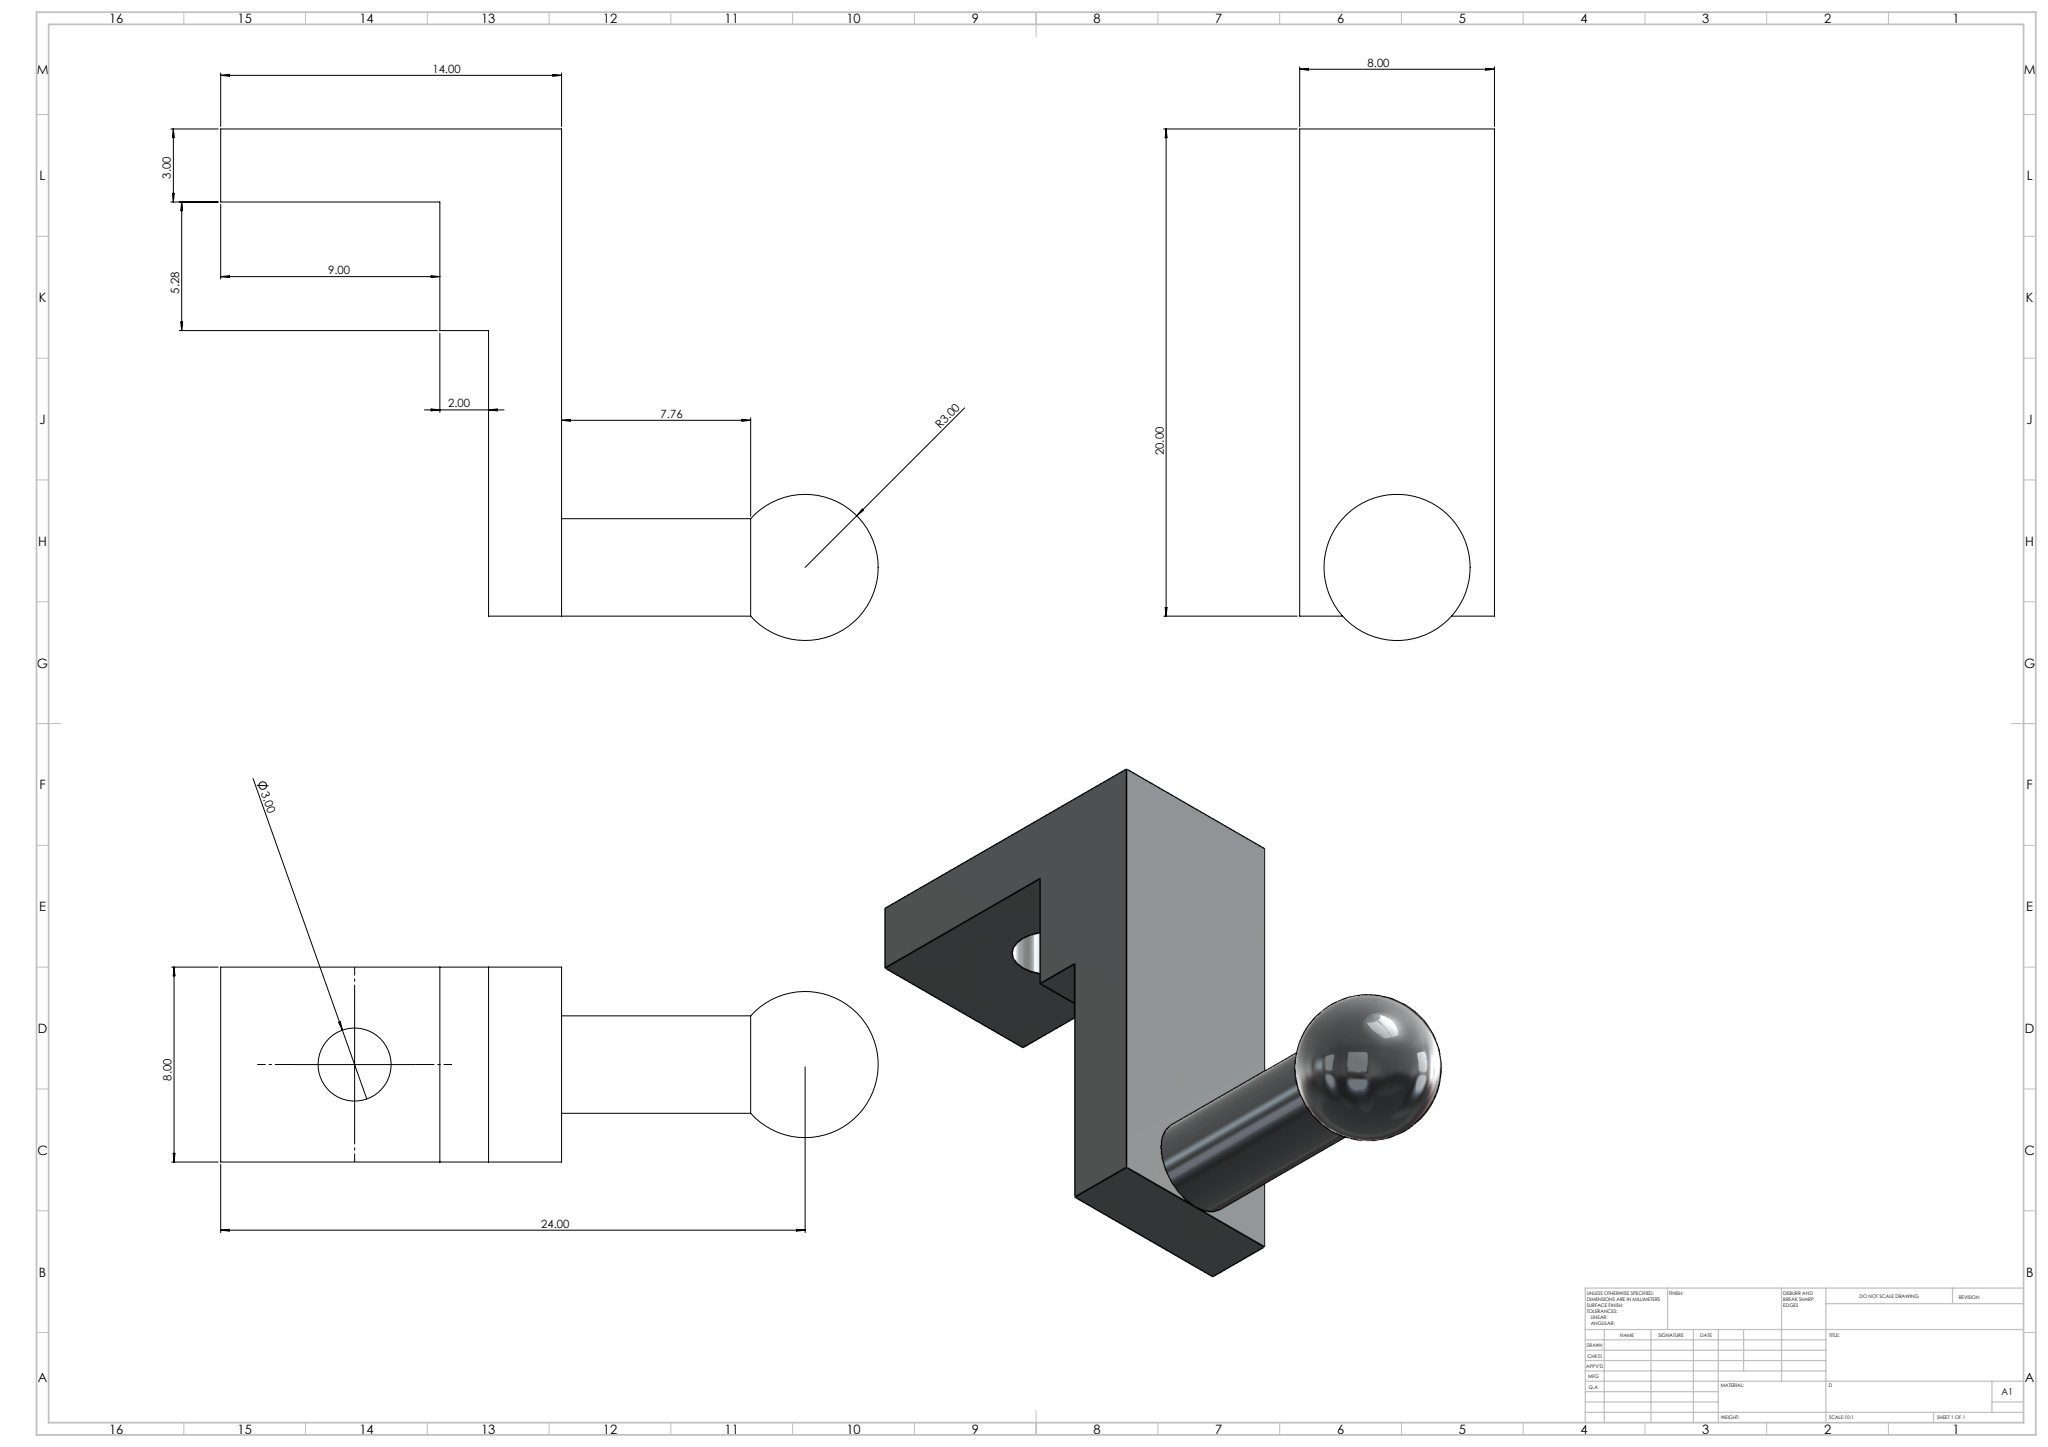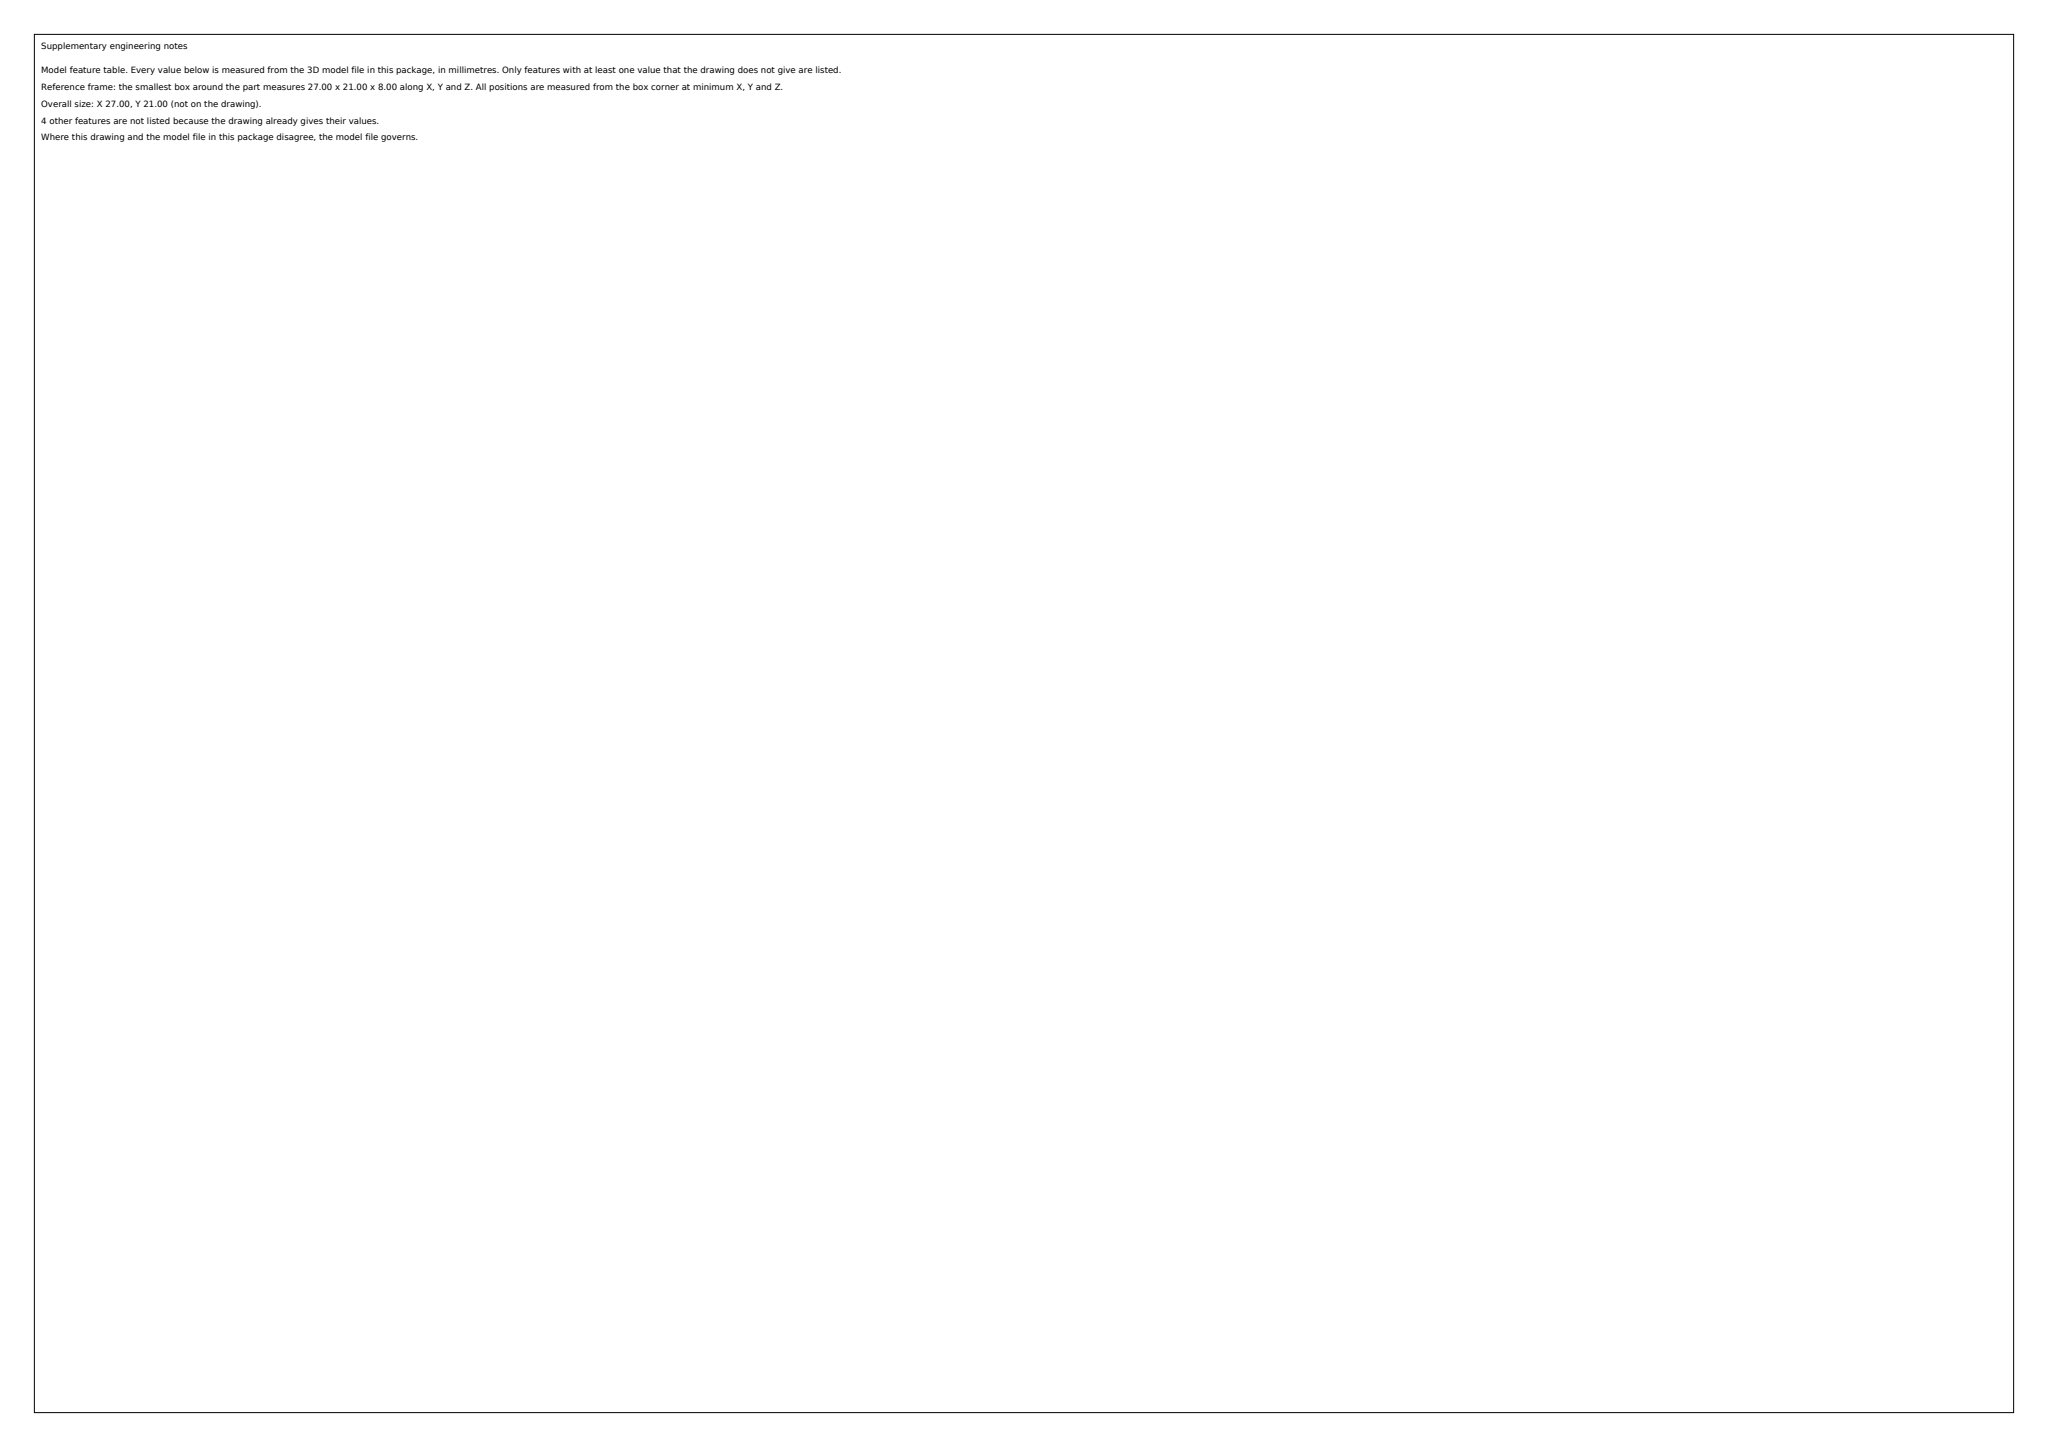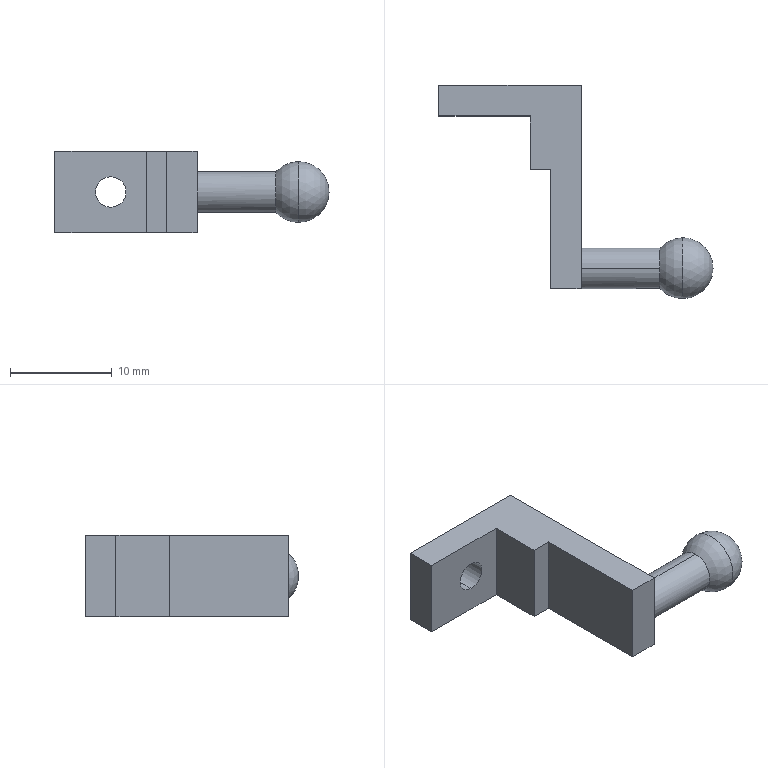Part | SolidWorks | mm | 1 solid | 16 faces | box 27 x 21 x 8 mm | volume 1013 mm3 | plane 10 | cylinder 4 | sphere 2 | commonest cylinder face diameters 3 x2 4 x2
build123d program:
from build123d import *

# Parameters (mm, degrees)
BOSS_EXTRUDE1_DEPTH = 8
SKETCH2_R           = 2
BOSS_EXTRUDE2_DEPTH = 10
CUT_EXTRUDE1_REACH  = 32.266
SKETCH4_R           = 1.5


with BuildPart() as part:
    # Sketch1 → Boss-Extrude1 (new body)
    with BuildSketch(Plane.XY):
        Polygon((-6.727, 7.437), (2.273, 7.437), (2.273, 2.159), (4.273, 2.159), (4.273, -9.563), (7.273, -9.563), (7.273, 10.437), (-6.727, 10.437), align=None)
    extrude(amount=BOSS_EXTRUDE1_DEPTH)

    # Sketch2 → Boss-Extrude2 (add)
    with BuildSketch(Plane(origin=(7.273, 0, 0), x_dir=(0, 0, -1), z_dir=(1, 0, 0))):
        with Locations(Location((-4, -7.563, 0), (0, 0, 270))):
            Circle(SKETCH2_R)
    extrude(amount=BOSS_EXTRUDE2_DEPTH)

    # Sketch3 → Revolve1 (revolve)
    with BuildSketch(Plane(origin=(17.273, 0, 0), x_dir=(0, 0, -1), z_dir=(1, 0, 0))):
        with BuildLine():
            Line((-7, -7.563), (-1, -7.563))
            ThreePointArc((-1, -7.563), (-4, -4.563), (-7, -7.563))
        make_face()
    revolve(axis=Axis((17.273, -7.563, 7), (0, 0, -1)))

    # Sketch4 → Cut-Extrude1 (cut, up to next)
    with BuildSketch(Plane(origin=(0, 10.437, 0), x_dir=(1, 0, 0), z_dir=(0, 1, 0)), mode=Mode.PRIVATE) as cut_extrude1_sk1:
        with Locations(Location((-1.227, -4, 0), (0, 0, 270))):
            Circle(SKETCH4_R)
    cut_extrude1_tool1 = extrude(cut_extrude1_sk1.sketch, amount=-CUT_EXTRUDE1_REACH, mode=Mode.PRIVATE) & part.part
    add(cut_extrude1_tool1.solids().sort_by_distance((-1.227, 10.437, 4))[0], mode=Mode.SUBTRACT)


solid = part.part
STEP:
#1=CARTESIAN_POINT('',(-1.227,7.437,5.5));
#2=VERTEX_POINT('',#1);
#3=CARTESIAN_POINT('',(-1.227,7.437,2.5));
#4=VERTEX_POINT('',#3);
#5=CARTESIAN_POINT('',(-1.227,7.437,4.));
#6=DIRECTION('',(0.,-1.,0.));
#7=DIRECTION('',(0.,0.,1.));
#8=AXIS2_PLACEMENT_3D('',#5,#6,#7);
#9=CIRCLE('',#8,1.5);
#10=EDGE_CURVE('',#2,#4,#9,.T.);
#11=ORIENTED_EDGE('',*,*,#10,.T.);
#12=CARTESIAN_POINT('',(-1.227,10.437,2.5));
#13=VERTEX_POINT('',#12);
#14=CARTESIAN_POINT('',(-1.227,-10.564,2.5));
#15=DIRECTION('',(0.,1.,0.));
#16=VECTOR('',#15,1000.);
#17=LINE('',#14,#16);
#18=EDGE_CURVE('',#4,#13,#17,.T.);
#19=ORIENTED_EDGE('',*,*,#18,.T.);
#20=CARTESIAN_POINT('',(-1.227,10.437,5.5));
#21=VERTEX_POINT('',#20);
#22=CARTESIAN_POINT('',(-1.227,10.437,4.));
#23=DIRECTION('',(0.,1.,0.));
#24=DIRECTION('',(0.,0.,1.));
#25=AXIS2_PLACEMENT_3D('',#22,#23,#24);
#26=CIRCLE('',#25,1.5);
#27=EDGE_CURVE('',#13,#21,#26,.T.);
#28=ORIENTED_EDGE('',*,*,#27,.T.);
#29=CARTESIAN_POINT('',(-1.227,-10.564,5.5));
#30=DIRECTION('',(0.,1.,0.));
#31=VECTOR('',#30,1000.);
#32=LINE('',#29,#31);
#33=EDGE_CURVE('',#2,#21,#32,.T.);
#34=ORIENTED_EDGE('',*,*,#33,.F.);
#35=EDGE_LOOP('',(#11,#19,#28,#34));
#36=FACE_OUTER_BOUND('',#35,.T.);
#37=CARTESIAN_POINT('',(-1.227,-10.564,4.));
#38=DIRECTION('',(0.,1.,0.));
#39=DIRECTION('',(0.,0.,1.));
#40=AXIS2_PLACEMENT_3D('',#37,#38,#39);
#41=CYLINDRICAL_SURFACE('',#40,1.5);
#42=ADVANCED_FACE('',(#36),#41,.F.);
#43=CARTESIAN_POINT('',(15.037,-7.563,6.));
#44=VERTEX_POINT('',#43);
#45=CARTESIAN_POINT('',(15.037,-7.563,2.));
#46=VERTEX_POINT('',#45);
#47=CARTESIAN_POINT('',(15.037,-7.563,4.));
#48=DIRECTION('',(1.,0.,0.));
#49=DIRECTION('',(0.,0.,-1.));
#50=AXIS2_PLACEMENT_3D('',#47,#48,#49);
#51=CIRCLE('',#50,2.);
#52=EDGE_CURVE('',#44,#46,#51,.T.);
#53=ORIENTED_EDGE('',*,*,#52,.T.);
#54=CARTESIAN_POINT('',(15.037,-7.563,4.));
#55=DIRECTION('',(1.,0.,0.));
#56=DIRECTION('',(0.,0.,-1.));
#57=AXIS2_PLACEMENT_3D('',#54,#55,#56);
#58=CIRCLE('',#57,2.);
#59=EDGE_CURVE('',#46,#44,#58,.T.);
#60=ORIENTED_EDGE('',*,*,#59,.T.);
#61=EDGE_LOOP('',(#53,#60));
#62=FACE_BOUND('',#61,.T.);
#63=CARTESIAN_POINT('',(17.273,-7.563,1.));
#64=VERTEX_POINT('',#63);
#65=CARTESIAN_POINT('',(17.273,-7.563,7.));
#66=VERTEX_POINT('',#65);
#67=CARTESIAN_POINT('',(17.273,-7.563,4.));
#68=DIRECTION('',(1.,0.,0.));
#69=DIRECTION('',(0.,0.,-1.));
#70=AXIS2_PLACEMENT_3D('',#67,#68,#69);
#71=CIRCLE('',#70,3.);
#72=EDGE_CURVE('',#64,#66,#71,.T.);
#73=ORIENTED_EDGE('',*,*,#72,.F.);
#74=CARTESIAN_POINT('',(17.273,-7.563,4.));
#75=DIRECTION('',(-1.,0.,0.));
#76=DIRECTION('',(0.,-1.,0.));
#77=AXIS2_PLACEMENT_3D('',#74,#75,#76);
#78=CIRCLE('',#77,3.);
#79=EDGE_CURVE('',#64,#66,#78,.T.);
#80=ORIENTED_EDGE('',*,*,#79,.T.);
#81=EDGE_LOOP('',(#73,#80));
#82=FACE_OUTER_BOUND('',#81,.T.);
#83=CARTESIAN_POINT('',(17.273,-7.563,4.));
#84=DIRECTION('',(-1.,0.,0.));
#85=DIRECTION('',(0.,1.,0.));
#86=AXIS2_PLACEMENT_3D('',#83,#84,#85);
#87=SPHERICAL_SURFACE('',#86,3.);
#88=ADVANCED_FACE('',(#62,#82),#87,.T.);
#89=ORIENTED_EDGE('',*,*,#59,.F.);
#90=CARTESIAN_POINT('',(7.273,-7.563,2.));
#91=VERTEX_POINT('',#90);
#92=CARTESIAN_POINT('',(17.273,-7.563,2.));
#93=DIRECTION('',(-1.,0.,0.));
#94=VECTOR('',#93,1000.);
#95=LINE('',#92,#94);
#96=EDGE_CURVE('',#46,#91,#95,.T.);
#97=ORIENTED_EDGE('',*,*,#96,.T.);
#98=CARTESIAN_POINT('',(7.273,-7.563,6.));
#99=VERTEX_POINT('',#98);
#100=CARTESIAN_POINT('',(7.273,-7.563,4.));
#101=DIRECTION('',(1.,0.,0.));
#102=DIRECTION('',(0.,0.,-1.));
#103=AXIS2_PLACEMENT_3D('',#100,#101,#102);
#104=CIRCLE('',#103,2.);
#105=EDGE_CURVE('',#91,#99,#104,.T.);
#106=ORIENTED_EDGE('',*,*,#105,.T.);
#107=CARTESIAN_POINT('',(17.273,-7.563,6.));
#108=DIRECTION('',(-1.,0.,0.));
#109=VECTOR('',#108,1000.);
#110=LINE('',#107,#109);
#111=EDGE_CURVE('',#44,#99,#110,.T.);
#112=ORIENTED_EDGE('',*,*,#111,.F.);
#113=EDGE_LOOP('',(#89,#97,#106,#112));
#114=FACE_OUTER_BOUND('',#113,.T.);
#115=CARTESIAN_POINT('',(17.273,-7.563,4.));
#116=DIRECTION('',(-1.,0.,0.));
#117=DIRECTION('',(0.,0.,1.));
#118=AXIS2_PLACEMENT_3D('',#115,#116,#117);
#119=CYLINDRICAL_SURFACE('',#118,2.);
#120=ADVANCED_FACE('',(#114),#119,.T.);
#121=ORIENTED_EDGE('',*,*,#96,.F.);
#122=ORIENTED_EDGE('',*,*,#52,.F.);
#123=ORIENTED_EDGE('',*,*,#111,.T.);
#124=CARTESIAN_POINT('',(7.273,-9.563,4.));
#125=VERTEX_POINT('',#124);
#126=CARTESIAN_POINT('',(7.273,-7.563,4.));
#127=DIRECTION('',(1.,0.,0.));
#128=DIRECTION('',(0.,0.,-1.));
#129=AXIS2_PLACEMENT_3D('',#126,#127,#128);
#130=CIRCLE('',#129,2.);
#131=EDGE_CURVE('',#99,#125,#130,.T.);
#132=ORIENTED_EDGE('',*,*,#131,.T.);
#133=CARTESIAN_POINT('',(7.273,-7.563,4.));
#134=DIRECTION('',(1.,0.,0.));
#135=DIRECTION('',(0.,0.,-1.));
#136=AXIS2_PLACEMENT_3D('',#133,#134,#135);
#137=CIRCLE('',#136,2.);
#138=EDGE_CURVE('',#125,#91,#137,.T.);
#139=ORIENTED_EDGE('',*,*,#138,.T.);
#140=EDGE_LOOP('',(#121,#122,#123,#132,#139));
#141=FACE_OUTER_BOUND('',#140,.T.);
#142=CARTESIAN_POINT('',(17.273,-7.563,4.));
#143=DIRECTION('',(-1.,0.,0.));
#144=DIRECTION('',(0.,0.,1.));
#145=AXIS2_PLACEMENT_3D('',#142,#143,#144);
#146=CYLINDRICAL_SURFACE('',#145,2.);
#147=ADVANCED_FACE('',(#141),#146,.T.);
#148=CARTESIAN_POINT('',(-6.727,10.437,0.));
#149=VERTEX_POINT('',#148);
#150=CARTESIAN_POINT('',(-6.727,7.437,0.));
#151=VERTEX_POINT('',#150);
#152=CARTESIAN_POINT('',(-6.727,10.437,0.));
#153=DIRECTION('',(0.,-1.,0.));
#154=VECTOR('',#153,1000.);
#155=LINE('',#152,#154);
#156=EDGE_CURVE('',#149,#151,#155,.T.);
#157=ORIENTED_EDGE('',*,*,#156,.T.);
#158=CARTESIAN_POINT('',(-6.727,7.437,8.));
#159=VERTEX_POINT('',#158);
#160=CARTESIAN_POINT('',(-6.727,7.437,8.));
#161=DIRECTION('',(0.,0.,-1.));
#162=VECTOR('',#161,1000.);
#163=LINE('',#160,#162);
#164=EDGE_CURVE('',#159,#151,#163,.T.);
#165=ORIENTED_EDGE('',*,*,#164,.F.);
#166=CARTESIAN_POINT('',(-6.727,10.437,8.));
#167=VERTEX_POINT('',#166);
#168=CARTESIAN_POINT('',(-6.727,10.437,8.));
#169=DIRECTION('',(0.,-1.,0.));
#170=VECTOR('',#169,1000.);
#171=LINE('',#168,#170);
#172=EDGE_CURVE('',#167,#159,#171,.T.);
#173=ORIENTED_EDGE('',*,*,#172,.F.);
#174=CARTESIAN_POINT('',(-6.727,10.437,8.));
#175=DIRECTION('',(0.,0.,-1.));
#176=VECTOR('',#175,1000.);
#177=LINE('',#174,#176);
#178=EDGE_CURVE('',#167,#149,#177,.T.);
#179=ORIENTED_EDGE('',*,*,#178,.T.);
#180=EDGE_LOOP('',(#157,#165,#173,#179));
#181=FACE_OUTER_BOUND('',#180,.T.);
#182=CARTESIAN_POINT('',(-6.727,10.437,8.));
#183=DIRECTION('',(1.,0.,0.));
#184=DIRECTION('',(0.,0.,-1.));
#185=AXIS2_PLACEMENT_3D('',#182,#183,#184);
#186=PLANE('',#185);
#187=ADVANCED_FACE('',(#181),#186,.F.);
#188=ORIENTED_EDGE('',*,*,#10,.F.);
#189=CARTESIAN_POINT('',(-1.227,7.437,4.));
#190=DIRECTION('',(0.,-1.,0.));
#191=DIRECTION('',(0.,0.,1.));
#192=AXIS2_PLACEMENT_3D('',#189,#190,#191);
#193=CIRCLE('',#192,1.5);
#194=EDGE_CURVE('',#4,#2,#193,.T.);
#195=ORIENTED_EDGE('',*,*,#194,.F.);
#196=EDGE_LOOP('',(#188,#195));
#197=FACE_BOUND('',#196,.T.);
#198=CARTESIAN_POINT('',(2.273,7.437,0.));
#199=VERTEX_POINT('',#198);
#200=CARTESIAN_POINT('',(-6.727,7.437,0.));
#201=DIRECTION('',(1.,0.,0.));
#202=VECTOR('',#201,1000.);
#203=LINE('',#200,#202);
#204=EDGE_CURVE('',#151,#199,#203,.T.);
#205=ORIENTED_EDGE('',*,*,#204,.T.);
#206=CARTESIAN_POINT('',(2.273,7.437,8.));
#207=VERTEX_POINT('',#206);
#208=CARTESIAN_POINT('',(2.273,7.437,8.));
#209=DIRECTION('',(0.,0.,-1.));
#210=VECTOR('',#209,1000.);
#211=LINE('',#208,#210);
#212=EDGE_CURVE('',#207,#199,#211,.T.);
#213=ORIENTED_EDGE('',*,*,#212,.F.);
#214=CARTESIAN_POINT('',(-6.727,7.437,8.));
#215=DIRECTION('',(1.,0.,0.));
#216=VECTOR('',#215,1000.);
#217=LINE('',#214,#216);
#218=EDGE_CURVE('',#159,#207,#217,.T.);
#219=ORIENTED_EDGE('',*,*,#218,.F.);
#220=ORIENTED_EDGE('',*,*,#164,.T.);
#221=EDGE_LOOP('',(#205,#213,#219,#220));
#222=FACE_OUTER_BOUND('',#221,.T.);
#223=CARTESIAN_POINT('',(-6.727,7.437,8.));
#224=DIRECTION('',(0.,1.,0.));
#225=DIRECTION('',(0.,0.,1.));
#226=AXIS2_PLACEMENT_3D('',#223,#224,#225);
#227=PLANE('',#226);
#228=ADVANCED_FACE('',(#197,#222),#227,.F.);
#229=CARTESIAN_POINT('',(2.273,2.159,0.));
#230=VERTEX_POINT('',#229);
#231=CARTESIAN_POINT('',(2.273,7.437,0.));
#232=DIRECTION('',(0.,-1.,0.));
#233=VECTOR('',#232,1000.);
#234=LINE('',#231,#233);
#235=EDGE_CURVE('',#199,#230,#234,.T.);
#236=ORIENTED_EDGE('',*,*,#235,.T.);
#237=CARTESIAN_POINT('',(2.273,2.159,8.));
#238=VERTEX_POINT('',#237);
#239=CARTESIAN_POINT('',(2.273,2.159,8.));
#240=DIRECTION('',(0.,0.,-1.));
#241=VECTOR('',#240,1000.);
#242=LINE('',#239,#241);
#243=EDGE_CURVE('',#238,#230,#242,.T.);
#244=ORIENTED_EDGE('',*,*,#243,.F.);
#245=CARTESIAN_POINT('',(2.273,7.437,8.));
#246=DIRECTION('',(0.,-1.,0.));
#247=VECTOR('',#246,1000.);
#248=LINE('',#245,#247);
#249=EDGE_CURVE('',#207,#238,#248,.T.);
#250=ORIENTED_EDGE('',*,*,#249,.F.);
#251=ORIENTED_EDGE('',*,*,#212,.T.);
#252=EDGE_LOOP('',(#236,#244,#250,#251));
#253=FACE_OUTER_BOUND('',#252,.T.);
#254=CARTESIAN_POINT('',(2.273,7.437,8.));
#255=DIRECTION('',(1.,0.,0.));
#256=DIRECTION('',(0.,0.,-1.));
#257=AXIS2_PLACEMENT_3D('',#254,#255,#256);
#258=PLANE('',#257);
#259=ADVANCED_FACE('',(#253),#258,.F.);
#260=CARTESIAN_POINT('',(4.273,2.159,0.));
#261=VERTEX_POINT('',#260);
#262=CARTESIAN_POINT('',(2.273,2.159,0.));
#263=DIRECTION('',(1.,0.,0.));
#264=VECTOR('',#263,1000.);
#265=LINE('',#262,#264);
#266=EDGE_CURVE('',#230,#261,#265,.T.);
#267=ORIENTED_EDGE('',*,*,#266,.T.);
#268=CARTESIAN_POINT('',(4.273,2.159,8.));
#269=VERTEX_POINT('',#268);
#270=CARTESIAN_POINT('',(4.273,2.159,8.));
#271=DIRECTION('',(0.,0.,-1.));
#272=VECTOR('',#271,1000.);
#273=LINE('',#270,#272);
#274=EDGE_CURVE('',#269,#261,#273,.T.);
#275=ORIENTED_EDGE('',*,*,#274,.F.);
#276=CARTESIAN_POINT('',(2.273,2.159,8.));
#277=DIRECTION('',(1.,0.,0.));
#278=VECTOR('',#277,1000.);
#279=LINE('',#276,#278);
#280=EDGE_CURVE('',#238,#269,#279,.T.);
#281=ORIENTED_EDGE('',*,*,#280,.F.);
#282=ORIENTED_EDGE('',*,*,#243,.T.);
#283=EDGE_LOOP('',(#267,#275,#281,#282));
#284=FACE_OUTER_BOUND('',#283,.T.);
#285=CARTESIAN_POINT('',(2.273,2.159,8.));
#286=DIRECTION('',(0.,1.,0.));
#287=DIRECTION('',(0.,0.,1.));
#288=AXIS2_PLACEMENT_3D('',#285,#286,#287);
#289=PLANE('',#288);
#290=ADVANCED_FACE('',(#284),#289,.F.);
#291=CARTESIAN_POINT('',(4.273,-9.563,0.));
#292=VERTEX_POINT('',#291);
#293=CARTESIAN_POINT('',(4.273,2.159,0.));
#294=DIRECTION('',(0.,-1.,0.));
#295=VECTOR('',#294,1000.);
#296=LINE('',#293,#295);
#297=EDGE_CURVE('',#261,#292,#296,.T.);
#298=ORIENTED_EDGE('',*,*,#297,.T.);
#299=CARTESIAN_POINT('',(4.273,-9.563,8.));
#300=VERTEX_POINT('',#299);
#301=CARTESIAN_POINT('',(4.273,-9.563,8.));
#302=DIRECTION('',(0.,0.,-1.));
#303=VECTOR('',#302,1000.);
#304=LINE('',#301,#303);
#305=EDGE_CURVE('',#300,#292,#304,.T.);
#306=ORIENTED_EDGE('',*,*,#305,.F.);
#307=CARTESIAN_POINT('',(4.273,2.159,8.));
#308=DIRECTION('',(0.,-1.,0.));
#309=VECTOR('',#308,1000.);
#310=LINE('',#307,#309);
#311=EDGE_CURVE('',#269,#300,#310,.T.);
#312=ORIENTED_EDGE('',*,*,#311,.F.);
#313=ORIENTED_EDGE('',*,*,#274,.T.);
#314=EDGE_LOOP('',(#298,#306,#312,#313));
#315=FACE_OUTER_BOUND('',#314,.T.);
#316=CARTESIAN_POINT('',(4.273,2.159,8.));
#317=DIRECTION('',(1.,0.,0.));
#318=DIRECTION('',(0.,0.,-1.));
#319=AXIS2_PLACEMENT_3D('',#316,#317,#318);
#320=PLANE('',#319);
#321=ADVANCED_FACE('',(#315),#320,.F.);
#322=CARTESIAN_POINT('',(7.273,-9.563,0.));
#323=VERTEX_POINT('',#322);
#324=CARTESIAN_POINT('',(4.273,-9.563,0.));
#325=DIRECTION('',(1.,0.,0.));
#326=VECTOR('',#325,1000.);
#327=LINE('',#324,#326);
#328=EDGE_CURVE('',#292,#323,#327,.T.);
#329=ORIENTED_EDGE('',*,*,#328,.T.);
#330=CARTESIAN_POINT('',(7.273,-9.563,8.));
#331=DIRECTION('',(0.,0.,-1.));
#332=VECTOR('',#331,1000.);
#333=LINE('',#330,#332);
#334=EDGE_CURVE('',#125,#323,#333,.T.);
#335=ORIENTED_EDGE('',*,*,#334,.F.);
#336=CARTESIAN_POINT('',(7.273,-9.563,8.));
#337=VERTEX_POINT('',#336);
#338=CARTESIAN_POINT('',(7.273,-9.563,8.));
#339=DIRECTION('',(0.,0.,-1.));
#340=VECTOR('',#339,1000.);
#341=LINE('',#338,#340);
#342=EDGE_CURVE('',#337,#125,#341,.T.);
#343=ORIENTED_EDGE('',*,*,#342,.F.);
#344=CARTESIAN_POINT('',(4.273,-9.563,8.));
#345=DIRECTION('',(1.,0.,0.));
#346=VECTOR('',#345,1000.);
#347=LINE('',#344,#346);
#348=EDGE_CURVE('',#300,#337,#347,.T.);
#349=ORIENTED_EDGE('',*,*,#348,.F.);
#350=ORIENTED_EDGE('',*,*,#305,.T.);
#351=EDGE_LOOP('',(#329,#335,#343,#349,#350));
#352=FACE_OUTER_BOUND('',#351,.T.);
#353=CARTESIAN_POINT('',(4.273,-9.563,8.));
#354=DIRECTION('',(0.,1.,0.));
#355=DIRECTION('',(0.,0.,1.));
#356=AXIS2_PLACEMENT_3D('',#353,#354,#355);
#357=PLANE('',#356);
#358=ADVANCED_FACE('',(#352),#357,.F.);
#359=ORIENTED_EDGE('',*,*,#342,.T.);
#360=ORIENTED_EDGE('',*,*,#131,.F.);
#361=ORIENTED_EDGE('',*,*,#105,.F.);
#362=ORIENTED_EDGE('',*,*,#138,.F.);
#363=ORIENTED_EDGE('',*,*,#334,.T.);
#364=CARTESIAN_POINT('',(7.273,10.437,0.));
#365=VERTEX_POINT('',#364);
#366=CARTESIAN_POINT('',(7.273,-9.563,0.));
#367=DIRECTION('',(0.,1.,0.));
#368=VECTOR('',#367,1000.);
#369=LINE('',#366,#368);
#370=EDGE_CURVE('',#323,#365,#369,.T.);
#371=ORIENTED_EDGE('',*,*,#370,.T.);
#372=CARTESIAN_POINT('',(7.273,10.437,8.));
#373=VERTEX_POINT('',#372);
#374=CARTESIAN_POINT('',(7.273,10.437,8.));
#375=DIRECTION('',(0.,0.,-1.));
#376=VECTOR('',#375,1000.);
#377=LINE('',#374,#376);
#378=EDGE_CURVE('',#373,#365,#377,.T.);
#379=ORIENTED_EDGE('',*,*,#378,.F.);
#380=CARTESIAN_POINT('',(7.273,-9.563,8.));
#381=DIRECTION('',(0.,1.,0.));
#382=VECTOR('',#381,1000.);
#383=LINE('',#380,#382);
#384=EDGE_CURVE('',#337,#373,#383,.T.);
#385=ORIENTED_EDGE('',*,*,#384,.F.);
#386=EDGE_LOOP('',(#359,#360,#361,#362,#363,#371,#379,#385));
#387=FACE_OUTER_BOUND('',#386,.T.);
#388=CARTESIAN_POINT('',(7.273,-9.563,8.));
#389=DIRECTION('',(-1.,0.,0.));
#390=DIRECTION('',(0.,0.,1.));
#391=AXIS2_PLACEMENT_3D('',#388,#389,#390);
#392=PLANE('',#391);
#393=ADVANCED_FACE('',(#387),#392,.F.);
#394=CARTESIAN_POINT('',(-1.227,10.437,4.));
#395=DIRECTION('',(0.,1.,0.));
#396=DIRECTION('',(0.,0.,1.));
#397=AXIS2_PLACEMENT_3D('',#394,#395,#396);
#398=CIRCLE('',#397,1.5);
#399=EDGE_CURVE('',#21,#13,#398,.T.);
#400=ORIENTED_EDGE('',*,*,#399,.F.);
#401=ORIENTED_EDGE('',*,*,#27,.F.);
#402=EDGE_LOOP('',(#400,#401));
#403=FACE_BOUND('',#402,.T.);
#404=CARTESIAN_POINT('',(7.273,10.437,0.));
#405=DIRECTION('',(-1.,0.,0.));
#406=VECTOR('',#405,1000.);
#407=LINE('',#404,#406);
#408=EDGE_CURVE('',#365,#149,#407,.T.);
#409=ORIENTED_EDGE('',*,*,#408,.T.);
#410=ORIENTED_EDGE('',*,*,#178,.F.);
#411=CARTESIAN_POINT('',(7.273,10.437,8.));
#412=DIRECTION('',(-1.,0.,0.));
#413=VECTOR('',#412,1000.);
#414=LINE('',#411,#413);
#415=EDGE_CURVE('',#373,#167,#414,.T.);
#416=ORIENTED_EDGE('',*,*,#415,.F.);
#417=ORIENTED_EDGE('',*,*,#378,.T.);
#418=EDGE_LOOP('',(#409,#410,#416,#417));
#419=FACE_OUTER_BOUND('',#418,.T.);
#420=CARTESIAN_POINT('',(7.273,10.437,8.));
#421=DIRECTION('',(0.,-1.,0.));
#422=DIRECTION('',(0.,0.,-1.));
#423=AXIS2_PLACEMENT_3D('',#420,#421,#422);
#424=PLANE('',#423);
#425=ADVANCED_FACE('',(#403,#419),#424,.F.);
#426=ORIENTED_EDGE('',*,*,#172,.T.);
#427=ORIENTED_EDGE('',*,*,#218,.T.);
#428=ORIENTED_EDGE('',*,*,#249,.T.);
#429=ORIENTED_EDGE('',*,*,#280,.T.);
#430=ORIENTED_EDGE('',*,*,#311,.T.);
#431=ORIENTED_EDGE('',*,*,#348,.T.);
#432=ORIENTED_EDGE('',*,*,#384,.T.);
#433=ORIENTED_EDGE('',*,*,#415,.T.);
#434=EDGE_LOOP('',(#426,#427,#428,#429,#430,#431,#432,#433));
#435=FACE_OUTER_BOUND('',#434,.T.);
#436=CARTESIAN_POINT('',(0.,0.,8.));
#437=DIRECTION('',(0.,0.,1.));
#438=DIRECTION('',(1.,0.,0.));
#439=AXIS2_PLACEMENT_3D('',#436,#437,#438);
#440=PLANE('',#439);
#441=ADVANCED_FACE('',(#435),#440,.T.);
#442=ORIENTED_EDGE('',*,*,#156,.F.);
#443=ORIENTED_EDGE('',*,*,#408,.F.);
#444=ORIENTED_EDGE('',*,*,#370,.F.);
#445=ORIENTED_EDGE('',*,*,#328,.F.);
#446=ORIENTED_EDGE('',*,*,#297,.F.);
#447=ORIENTED_EDGE('',*,*,#266,.F.);
#448=ORIENTED_EDGE('',*,*,#235,.F.);
#449=ORIENTED_EDGE('',*,*,#204,.F.);
#450=EDGE_LOOP('',(#442,#443,#444,#445,#446,#447,#448,#449));
#451=FACE_OUTER_BOUND('',#450,.T.);
#452=CARTESIAN_POINT('',(0.,0.,0.));
#453=DIRECTION('',(0.,0.,1.));
#454=DIRECTION('',(1.,0.,0.));
#455=AXIS2_PLACEMENT_3D('',#452,#453,#454);
#456=PLANE('',#455);
#457=ADVANCED_FACE('',(#451),#456,.F.);
#458=ORIENTED_EDGE('',*,*,#79,.F.);
#459=ORIENTED_EDGE('',*,*,#72,.T.);
#460=EDGE_LOOP('',(#458,#459));
#461=FACE_OUTER_BOUND('',#460,.T.);
#462=CARTESIAN_POINT('',(17.273,-7.563,4.));
#463=DIRECTION('',(-1.,0.,0.));
#464=DIRECTION('',(0.,1.,0.));
#465=AXIS2_PLACEMENT_3D('',#462,#463,#464);
#466=SPHERICAL_SURFACE('',#465,3.);
#467=ADVANCED_FACE('',(#461),#466,.T.);
#468=ORIENTED_EDGE('',*,*,#18,.F.);
#469=ORIENTED_EDGE('',*,*,#194,.T.);
#470=ORIENTED_EDGE('',*,*,#33,.T.);
#471=ORIENTED_EDGE('',*,*,#399,.T.);
#472=EDGE_LOOP('',(#468,#469,#470,#471));
#473=FACE_OUTER_BOUND('',#472,.T.);
#474=CARTESIAN_POINT('',(-1.227,-10.564,4.));
#475=DIRECTION('',(0.,1.,0.));
#476=DIRECTION('',(0.,0.,1.));
#477=AXIS2_PLACEMENT_3D('',#474,#475,#476);
#478=CYLINDRICAL_SURFACE('',#477,1.5);
#479=ADVANCED_FACE('',(#473),#478,.F.);
#480=CLOSED_SHELL('',(#42,#88,#120,#147,#187,#228,#259,#290,#321,#358,#393,#425,#441,#457,#467,#479));
#481=MANIFOLD_SOLID_BREP('',#480);
#482=CARTESIAN_POINT('',(0.,0.,0.));
#483=DIRECTION('',(0.,0.,1.));
#484=DIRECTION('',(1.,0.,0.));
#485=AXIS2_PLACEMENT_3D('',#482,#483,#484);
#486=(LENGTH_UNIT()NAMED_UNIT(*)SI_UNIT(.MILLI.,.METRE.));
#487=UNCERTAINTY_MEASURE_WITH_UNIT(LENGTH_MEASURE(0.00001),#486,'','');
#488=(NAMED_UNIT(*)PLANE_ANGLE_UNIT()SI_UNIT($,.RADIAN.));
#489=(NAMED_UNIT(*)SI_UNIT($,.STERADIAN.)SOLID_ANGLE_UNIT());
#490=(GEOMETRIC_REPRESENTATION_CONTEXT(3)GLOBAL_UNCERTAINTY_ASSIGNED_CONTEXT((#487))GLOBAL_UNIT_ASSIGNED_CONTEXT((#486,#488,#489))REPRESENTATION_CONTEXT('',''));
#491=ADVANCED_BREP_SHAPE_REPRESENTATION('',(#481,#485),#490);